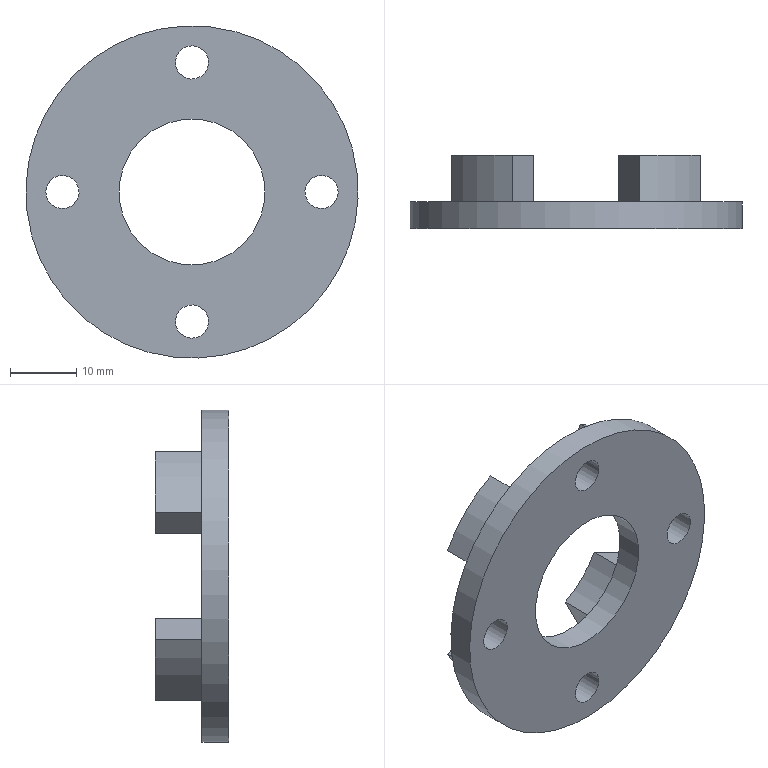Component | NX | COVER | 1 solid | 28 faces | volume 8174 mm3 | cylinder 14 | plane 14 | commonest cylinder face diameters 5 x4 28 x4 42 x4 22 x1 50 x1